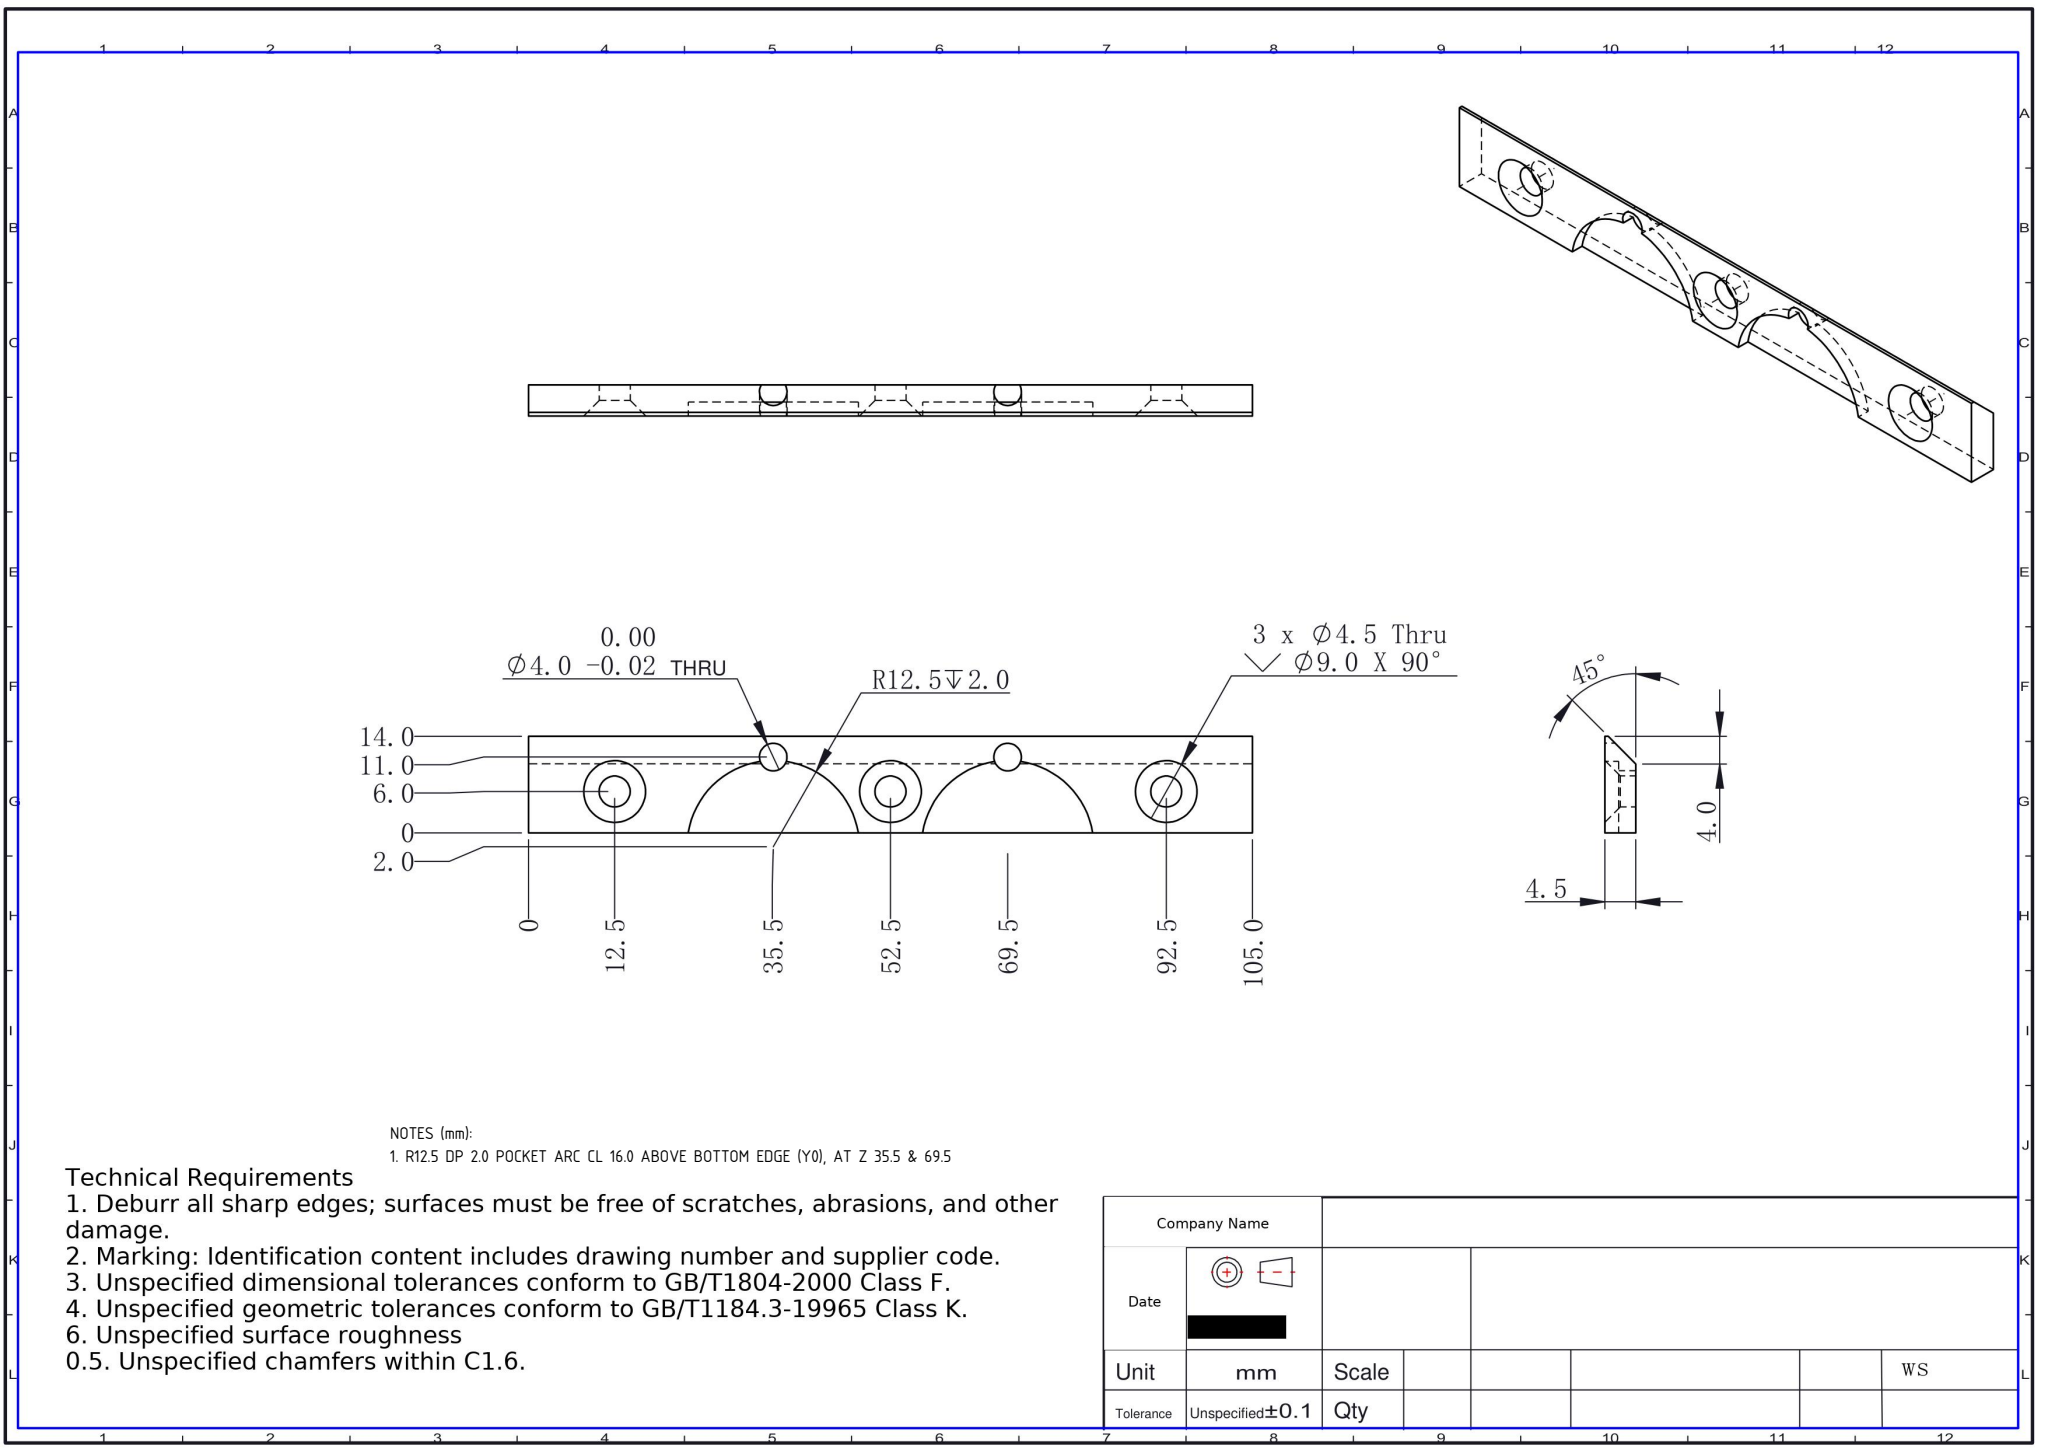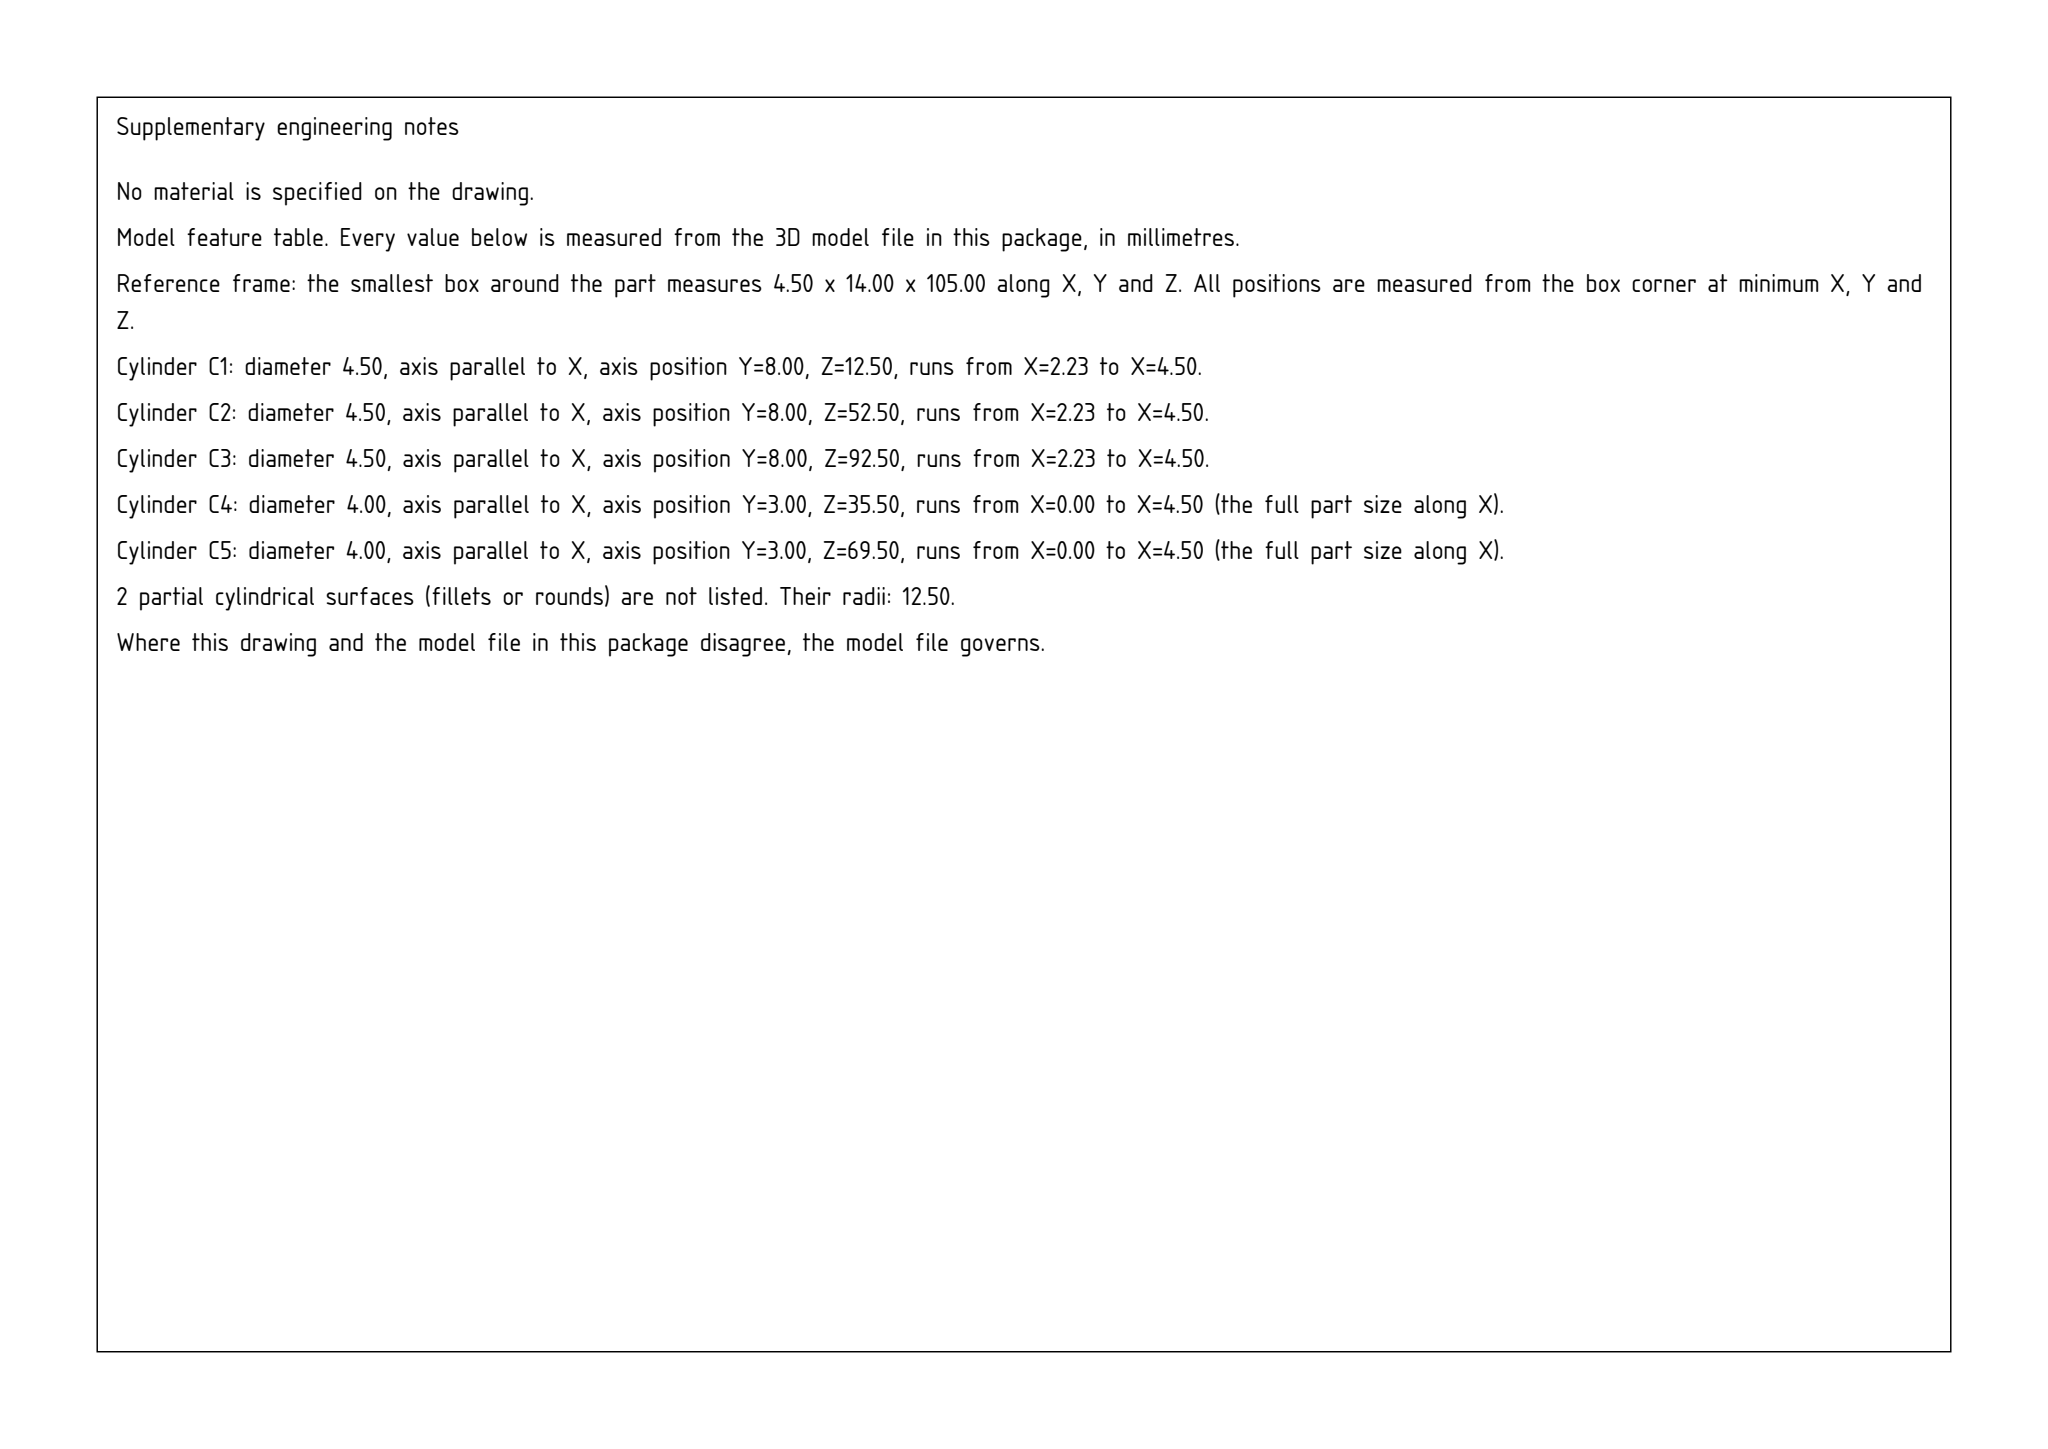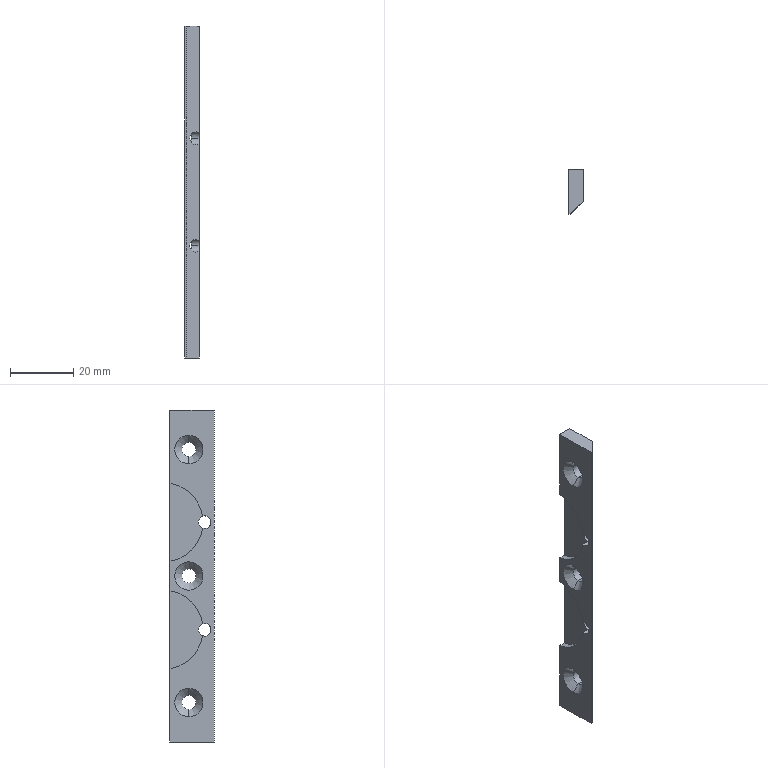Part | SolidWorks | mm | 1 solid | 29 faces | box 4.5 x 14 x 105 mm | volume 4568 mm3 | cylinder 14 | plane 9 | cone 6 | commonest cylinder face diameters 4.5 x6 4 x4 25 x4
Drawing notes:
R12.5 DP 2.0 POCKET ARC CL 16.0 ABOVE BOTTOM EDGE (Y0), AT Z 35.5 & 69.5 | from the solid: cylinders dia 25.0 axis x at [y=16.0, z=35.5] and [y=16.0, z=69.5], depth 2.0; part Y extent 0 to 14.0
build123d program:
from build123d import *

# Parameters (mm, degrees)
BOSS_EXTRUDE1_DEPTH                                  = 105
COUNTERSUNK_HOLE_1_FOR_M4_HEXAGON_SOCKET_D           = 4.5
COUNTERSUNK_HOLE_1_FOR_M4_HEXAGON_SOCKET_CSINK_D     = 8.96
COUNTERSUNK_HOLE_1_FOR_M4_HEXAGON_SOCKET_CSINK_ANGLE = 90
SKETCH5_R                                            = 12.5
CUT_EXTRUDE1_DEPTH                                   = 2
SKETCH6_R                                            = 2
CUT_EXTRUDE2_DEPTH                                   = 107.025


with BuildPart() as part:
    # Sketch1 → Boss-Extrude1 (new body)
    with BuildSketch(Plane.XY):
        Polygon((4.5, -10), (0.5, -14), (0, -14), (0, 0), (4.5, 0), align=None)
    extrude(amount=BOSS_EXTRUDE1_DEPTH)

    # Countersunk Hole 1 for M4 Hexagon Socket (through all)
    with Locations(Plane.ZY):
        with Locations((12.5, -6), (92.5, -6), (52.5, -6)):
            CounterSinkHole(COUNTERSUNK_HOLE_1_FOR_M4_HEXAGON_SOCKET_D / 2, COUNTERSUNK_HOLE_1_FOR_M4_HEXAGON_SOCKET_CSINK_D / 2, counter_sink_angle=COUNTERSUNK_HOLE_1_FOR_M4_HEXAGON_SOCKET_CSINK_ANGLE)

    # Sketch5 → Cut-Extrude1 (cut)
    with BuildSketch(Plane.ZY):
        with Locations((69.5, 2)):
            Circle(SKETCH5_R)
        with Locations((35.5, 2)):
            Circle(SKETCH5_R)
    extrude(amount=-CUT_EXTRUDE1_DEPTH, mode=Mode.SUBTRACT)

    # Sketch6 → Cut-Extrude2 (cut, through all)
    with BuildSketch(Plane(origin=(4.5, 0, 0), x_dir=(0, 0, -1), z_dir=(1, 0, 0))):
        with Locations(Location((-69.5, -11, 0), (0, 0, 30))):
            Circle(SKETCH6_R)
        with Locations(Location((-35.5, -11, 0), (0, 0, 150))):
            Circle(SKETCH6_R)
    extrude(amount=-CUT_EXTRUDE2_DEPTH, mode=Mode.SUBTRACT)


solid = part.part